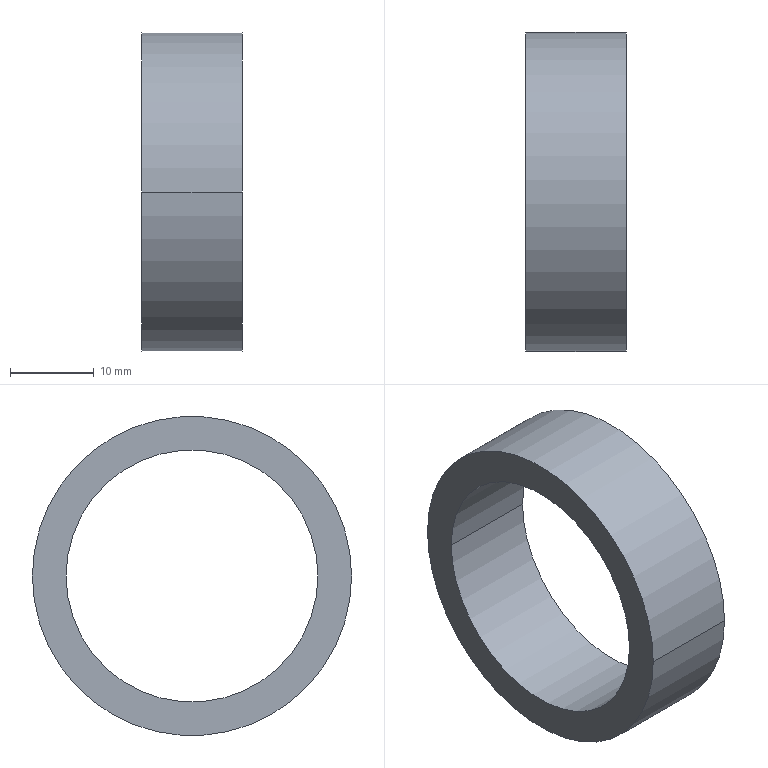Component | SolidWorks | LowerSideBeltXG-XG1-1_DriveShaftSpacerXG-XG1-1 | 1 solid | 6 faces | box 12 x 38 x 38 mm | volume 5127 mm3 | cylinder 4 | plane 2 | commonest cylinder face diameters 30 x2 38 x2
build123d program:
from build123d import *

# Parameters (mm, degrees)
SKETCH1_R           = 19
SKETCH1_R_2         = 15
BOSS_EXTRUDE1_DEPTH = 6


with BuildPart() as part:
    # Sketch1 → Boss-Extrude1 (new, symmetric)
    with BuildSketch(Plane(origin=(0, 0, 0), x_dir=(0, 0, -1), z_dir=(1, 0, 0))):
        Circle(SKETCH1_R)
        Circle(SKETCH1_R_2, mode=Mode.SUBTRACT)
    extrude(amount=BOSS_EXTRUDE1_DEPTH, both=True)


solid = part.part

# Placed as in the assembly
solid = solid.moved(Location((-297.22, 625, 114), (0, 0, 0)))
STEP:
#1=COLOUR_RGB('',0.7922,0.8196,0.9333);
#2=FILL_AREA_STYLE_COLOUR('',#1);
#3=FILL_AREA_STYLE('',(#2));
#4=SURFACE_STYLE_FILL_AREA(#3);
#5=SURFACE_SIDE_STYLE('',(#4));
#6=SURFACE_STYLE_USAGE(.BOTH.,#5);
#7=PRESENTATION_STYLE_ASSIGNMENT((#6));
#8=CARTESIAN_POINT('',(-11.465,24.016,4.488));
#9=VERTEX_POINT('',#8);
#10=CARTESIAN_POINT('',(-11.465,25.197,4.488));
#11=VERTEX_POINT('',#10);
#12=CARTESIAN_POINT('',(-11.465,24.606,4.488));
#13=DIRECTION('',(1.,0.,-0.));
#14=DIRECTION('',(0.,1.,0.));
#15=AXIS2_PLACEMENT_3D('',#12,#13,#14);
#16=CIRCLE('',#15,0.5906);
#17=EDGE_CURVE('',#9,#11,#16,.T.);
#18=ORIENTED_EDGE('',*,*,#17,.T.);
#19=CARTESIAN_POINT('',(-11.938,25.197,4.488));
#20=VERTEX_POINT('',#19);
#21=CARTESIAN_POINT('',(-11.465,25.197,4.488));
#22=DIRECTION('',(-1.,-0.,0.));
#23=VECTOR('',#22,39.37);
#24=LINE('',#21,#23);
#25=EDGE_CURVE('',#11,#20,#24,.T.);
#26=ORIENTED_EDGE('',*,*,#25,.T.);
#27=CARTESIAN_POINT('',(-11.938,24.016,4.488));
#28=VERTEX_POINT('',#27);
#29=CARTESIAN_POINT('',(-11.938,24.606,4.488));
#30=DIRECTION('',(1.,0.,-0.));
#31=DIRECTION('',(0.,1.,0.));
#32=AXIS2_PLACEMENT_3D('',#29,#30,#31);
#33=CIRCLE('',#32,0.5906);
#34=EDGE_CURVE('',#28,#20,#33,.T.);
#35=ORIENTED_EDGE('',*,*,#34,.F.);
#36=CARTESIAN_POINT('',(-11.465,24.016,4.488));
#37=DIRECTION('',(-1.,-0.,0.));
#38=VECTOR('',#37,39.37);
#39=LINE('',#36,#38);
#40=EDGE_CURVE('',#9,#28,#39,.T.);
#41=ORIENTED_EDGE('',*,*,#40,.F.);
#42=EDGE_LOOP('',(#18,#26,#35,#41));
#43=FACE_OUTER_BOUND('',#42,.T.);
#44=CARTESIAN_POINT('',(-11.465,24.606,4.488));
#45=DIRECTION('',(-1.,-0.,0.));
#46=DIRECTION('',(0.,-1.,0.));
#47=AXIS2_PLACEMENT_3D('',#44,#45,#46);
#48=CYLINDRICAL_SURFACE('',#47,0.5906);
#49=ADVANCED_FACE('',(#43),#48,.F.);
#50=CARTESIAN_POINT('',(-11.465,25.354,4.488));
#51=VERTEX_POINT('',#50);
#52=CARTESIAN_POINT('',(-11.465,23.858,4.488));
#53=VERTEX_POINT('',#52);
#54=CARTESIAN_POINT('',(-11.465,24.606,4.488));
#55=DIRECTION('',(1.,0.,-0.));
#56=DIRECTION('',(0.,1.,0.));
#57=AXIS2_PLACEMENT_3D('',#54,#55,#56);
#58=CIRCLE('',#57,0.748);
#59=EDGE_CURVE('',#51,#53,#58,.T.);
#60=ORIENTED_EDGE('',*,*,#59,.F.);
#61=CARTESIAN_POINT('',(-11.938,25.354,4.488));
#62=VERTEX_POINT('',#61);
#63=CARTESIAN_POINT('',(-11.465,25.354,4.488));
#64=DIRECTION('',(-1.,-0.,0.));
#65=VECTOR('',#64,39.37);
#66=LINE('',#63,#65);
#67=EDGE_CURVE('',#51,#62,#66,.T.);
#68=ORIENTED_EDGE('',*,*,#67,.T.);
#69=CARTESIAN_POINT('',(-11.938,23.858,4.488));
#70=VERTEX_POINT('',#69);
#71=CARTESIAN_POINT('',(-11.938,24.606,4.488));
#72=DIRECTION('',(1.,0.,-0.));
#73=DIRECTION('',(0.,1.,0.));
#74=AXIS2_PLACEMENT_3D('',#71,#72,#73);
#75=CIRCLE('',#74,0.748);
#76=EDGE_CURVE('',#62,#70,#75,.T.);
#77=ORIENTED_EDGE('',*,*,#76,.T.);
#78=CARTESIAN_POINT('',(-11.465,23.858,4.488));
#79=DIRECTION('',(-1.,-0.,0.));
#80=VECTOR('',#79,39.37);
#81=LINE('',#78,#80);
#82=EDGE_CURVE('',#53,#70,#81,.T.);
#83=ORIENTED_EDGE('',*,*,#82,.F.);
#84=EDGE_LOOP('',(#60,#68,#77,#83));
#85=FACE_OUTER_BOUND('',#84,.T.);
#86=CARTESIAN_POINT('',(-11.465,24.606,4.488));
#87=DIRECTION('',(-1.,-0.,0.));
#88=DIRECTION('',(0.,-1.,0.));
#89=AXIS2_PLACEMENT_3D('',#86,#87,#88);
#90=CYLINDRICAL_SURFACE('',#89,0.748);
#91=ADVANCED_FACE('',(#85),#90,.T.);
#92=CARTESIAN_POINT('',(-11.465,24.606,4.488));
#93=DIRECTION('',(1.,0.,-0.));
#94=DIRECTION('',(0.,1.,0.));
#95=AXIS2_PLACEMENT_3D('',#92,#93,#94);
#96=CIRCLE('',#95,0.748);
#97=EDGE_CURVE('',#53,#51,#96,.T.);
#98=ORIENTED_EDGE('',*,*,#97,.T.);
#99=ORIENTED_EDGE('',*,*,#59,.T.);
#100=EDGE_LOOP('',(#98,#99));
#101=FACE_OUTER_BOUND('',#100,.T.);
#102=ORIENTED_EDGE('',*,*,#17,.F.);
#103=CARTESIAN_POINT('',(-11.465,24.606,4.488));
#104=DIRECTION('',(1.,0.,-0.));
#105=DIRECTION('',(0.,1.,0.));
#106=AXIS2_PLACEMENT_3D('',#103,#104,#105);
#107=CIRCLE('',#106,0.5906);
#108=EDGE_CURVE('',#11,#9,#107,.T.);
#109=ORIENTED_EDGE('',*,*,#108,.F.);
#110=EDGE_LOOP('',(#102,#109));
#111=FACE_BOUND('',#110,.T.);
#112=CARTESIAN_POINT('',(-11.465,24.606,4.488));
#113=DIRECTION('',(1.,0.,-0.));
#114=DIRECTION('',(-0.,1.,0.));
#115=AXIS2_PLACEMENT_3D('',#112,#113,#114);
#116=PLANE('',#115);
#117=ADVANCED_FACE('',(#101,#111),#116,.T.);
#118=CARTESIAN_POINT('',(-11.938,24.606,4.488));
#119=DIRECTION('',(1.,0.,-0.));
#120=DIRECTION('',(0.,1.,0.));
#121=AXIS2_PLACEMENT_3D('',#118,#119,#120);
#122=CIRCLE('',#121,0.748);
#123=EDGE_CURVE('',#70,#62,#122,.T.);
#124=ORIENTED_EDGE('',*,*,#123,.F.);
#125=ORIENTED_EDGE('',*,*,#76,.F.);
#126=EDGE_LOOP('',(#124,#125));
#127=FACE_OUTER_BOUND('',#126,.T.);
#128=ORIENTED_EDGE('',*,*,#34,.T.);
#129=CARTESIAN_POINT('',(-11.938,24.606,4.488));
#130=DIRECTION('',(1.,0.,-0.));
#131=DIRECTION('',(0.,1.,0.));
#132=AXIS2_PLACEMENT_3D('',#129,#130,#131);
#133=CIRCLE('',#132,0.5906);
#134=EDGE_CURVE('',#20,#28,#133,.T.);
#135=ORIENTED_EDGE('',*,*,#134,.T.);
#136=EDGE_LOOP('',(#128,#135));
#137=FACE_BOUND('',#136,.T.);
#138=CARTESIAN_POINT('',(-11.938,24.606,4.488));
#139=DIRECTION('',(1.,0.,-0.));
#140=DIRECTION('',(-0.,1.,0.));
#141=AXIS2_PLACEMENT_3D('',#138,#139,#140);
#142=PLANE('',#141);
#143=ADVANCED_FACE('',(#127,#137),#142,.F.);
#144=ORIENTED_EDGE('',*,*,#67,.F.);
#145=ORIENTED_EDGE('',*,*,#97,.F.);
#146=ORIENTED_EDGE('',*,*,#82,.T.);
#147=ORIENTED_EDGE('',*,*,#123,.T.);
#148=EDGE_LOOP('',(#144,#145,#146,#147));
#149=FACE_OUTER_BOUND('',#148,.T.);
#150=CARTESIAN_POINT('',(-11.465,24.606,4.488));
#151=DIRECTION('',(-1.,-0.,0.));
#152=DIRECTION('',(0.,-1.,0.));
#153=AXIS2_PLACEMENT_3D('',#150,#151,#152);
#154=CYLINDRICAL_SURFACE('',#153,0.748);
#155=ADVANCED_FACE('',(#149),#154,.T.);
#156=ORIENTED_EDGE('',*,*,#25,.F.);
#157=ORIENTED_EDGE('',*,*,#108,.T.);
#158=ORIENTED_EDGE('',*,*,#40,.T.);
#159=ORIENTED_EDGE('',*,*,#134,.F.);
#160=EDGE_LOOP('',(#156,#157,#158,#159));
#161=FACE_OUTER_BOUND('',#160,.T.);
#162=CARTESIAN_POINT('',(-11.465,24.606,4.488));
#163=DIRECTION('',(-1.,-0.,0.));
#164=DIRECTION('',(0.,-1.,0.));
#165=AXIS2_PLACEMENT_3D('',#162,#163,#164);
#166=CYLINDRICAL_SURFACE('',#165,0.5906);
#167=ADVANCED_FACE('',(#161),#166,.F.);
#168=CLOSED_SHELL('',(#49,#91,#117,#143,#155,#167));
#169=MANIFOLD_SOLID_BREP('',#168);
#170=STYLED_ITEM('',(#7),#169);
#171=PRESENTATION_LAYER_ASSIGNMENT('','',(#170));
#172=CARTESIAN_POINT('',(0.,0.,0.));
#173=DIRECTION('',(0.,0.,1.));
#174=DIRECTION('',(1.,0.,0.));
#175=AXIS2_PLACEMENT_3D('',#172,#173,#174);
#176=(LENGTH_UNIT()NAMED_UNIT(*)SI_UNIT($,.METRE.));
#177=LENGTH_MEASURE_WITH_UNIT(LENGTH_MEASURE(0.0254),#176);
#178=DIMENSIONAL_EXPONENTS(1.,0.,0.,0.,0.,0.,0.);
#179=(CONVERSION_BASED_UNIT('',#177)LENGTH_UNIT()NAMED_UNIT(#178));
#180=UNCERTAINTY_MEASURE_WITH_UNIT(LENGTH_MEASURE(0.00001),#179,'','');
#181=(NAMED_UNIT(*)PLANE_ANGLE_UNIT()SI_UNIT($,.RADIAN.));
#182=(NAMED_UNIT(*)SI_UNIT($,.STERADIAN.)SOLID_ANGLE_UNIT());
#183=(GEOMETRIC_REPRESENTATION_CONTEXT(3)GLOBAL_UNCERTAINTY_ASSIGNED_CONTEXT((#180))GLOBAL_UNIT_ASSIGNED_CONTEXT((#179,#181,#182))REPRESENTATION_CONTEXT('',''));
#184=ADVANCED_BREP_SHAPE_REPRESENTATION('',(#169,#175),#183);
#185=(LENGTH_UNIT()NAMED_UNIT(*)SI_UNIT($,.METRE.));
#186=LENGTH_MEASURE_WITH_UNIT(LENGTH_MEASURE(0.0254),#185);
#187=DIMENSIONAL_EXPONENTS(1.,0.,0.,0.,0.,0.,0.);
#188=(CONVERSION_BASED_UNIT('',#186)LENGTH_UNIT()NAMED_UNIT(#187));
#189=UNCERTAINTY_MEASURE_WITH_UNIT(LENGTH_MEASURE(0.00001),#188,'','');
#190=(NAMED_UNIT(*)PLANE_ANGLE_UNIT()SI_UNIT($,.RADIAN.));
#191=(NAMED_UNIT(*)SI_UNIT($,.STERADIAN.)SOLID_ANGLE_UNIT());
#192=(GEOMETRIC_REPRESENTATION_CONTEXT(3)GLOBAL_UNCERTAINTY_ASSIGNED_CONTEXT((#189))GLOBAL_UNIT_ASSIGNED_CONTEXT((#188,#190,#191))REPRESENTATION_CONTEXT('',''));
#193=MECHANICAL_DESIGN_GEOMETRIC_PRESENTATION_REPRESENTATION('',(#170),#192);